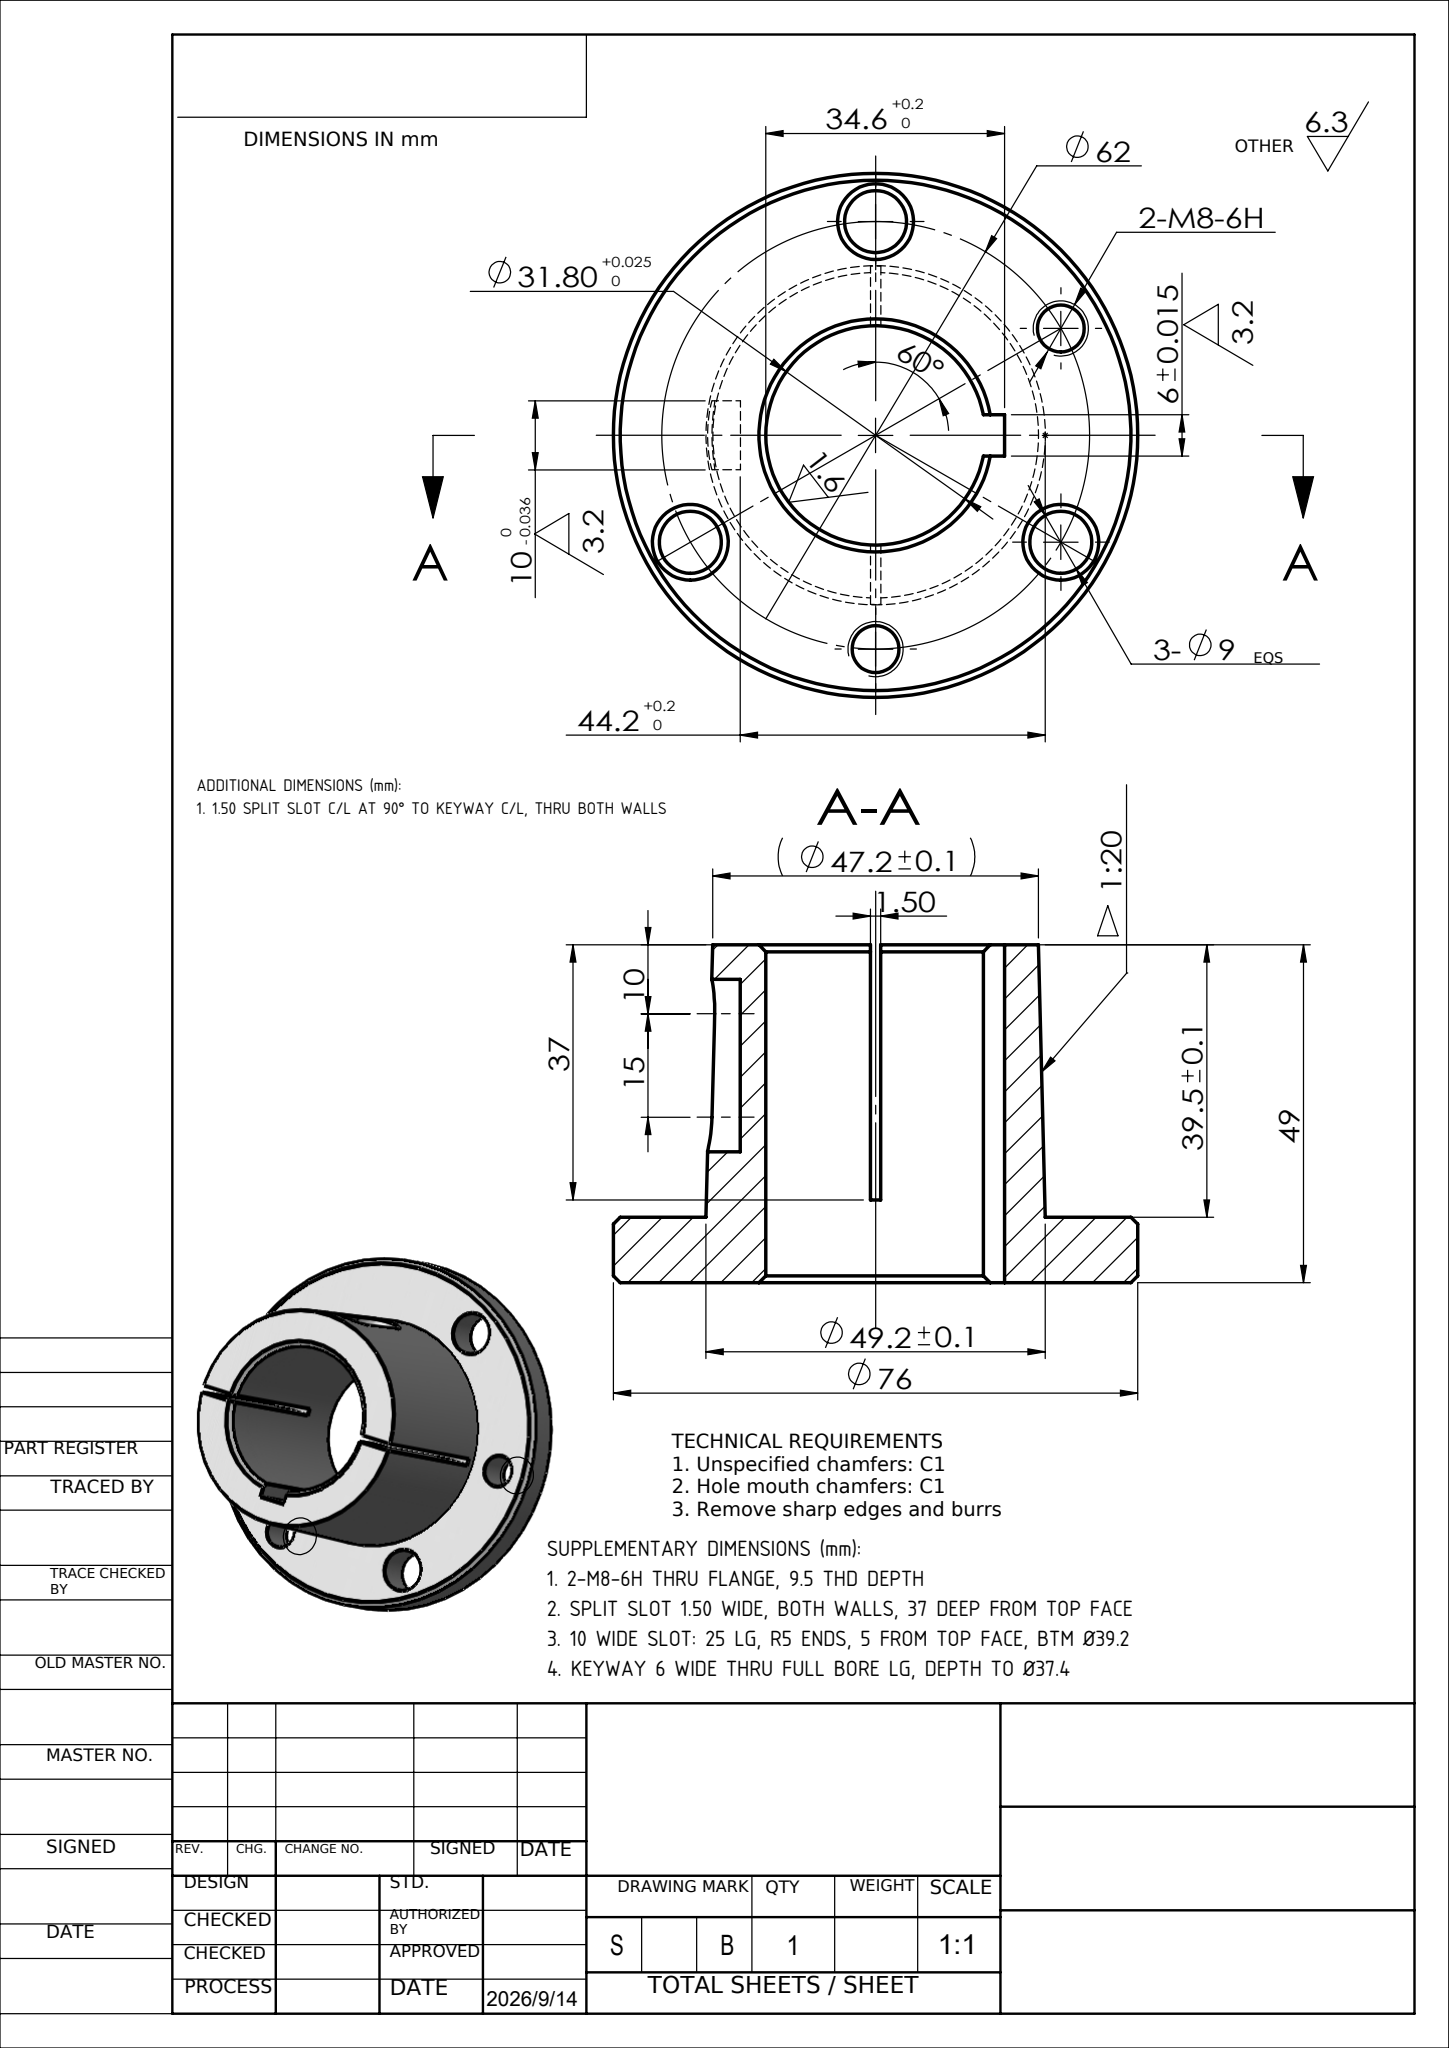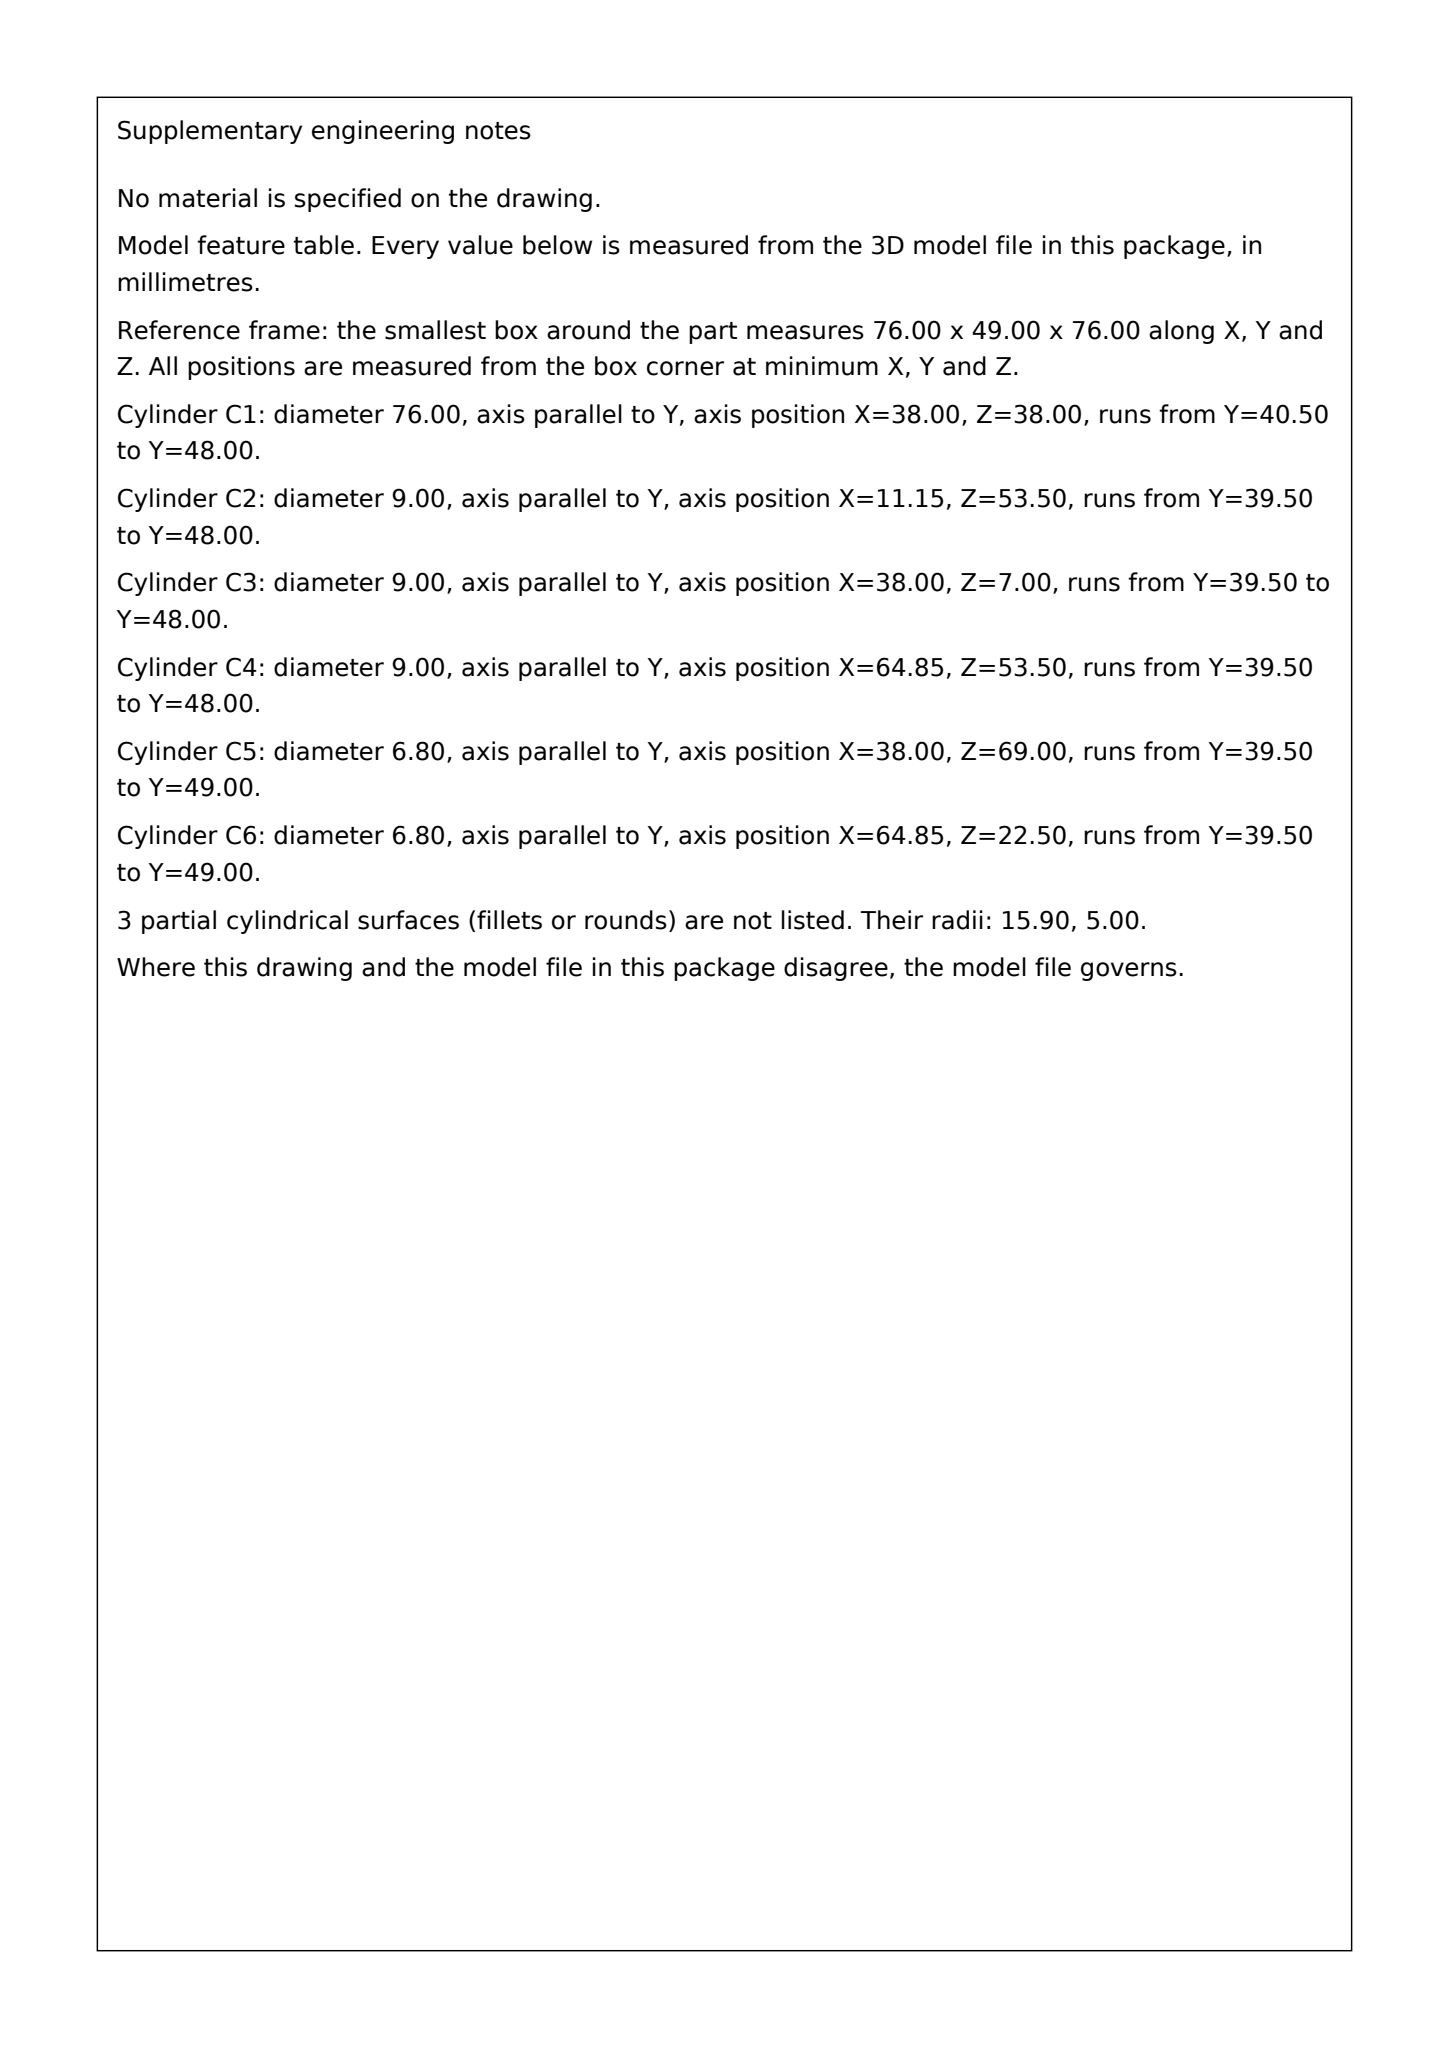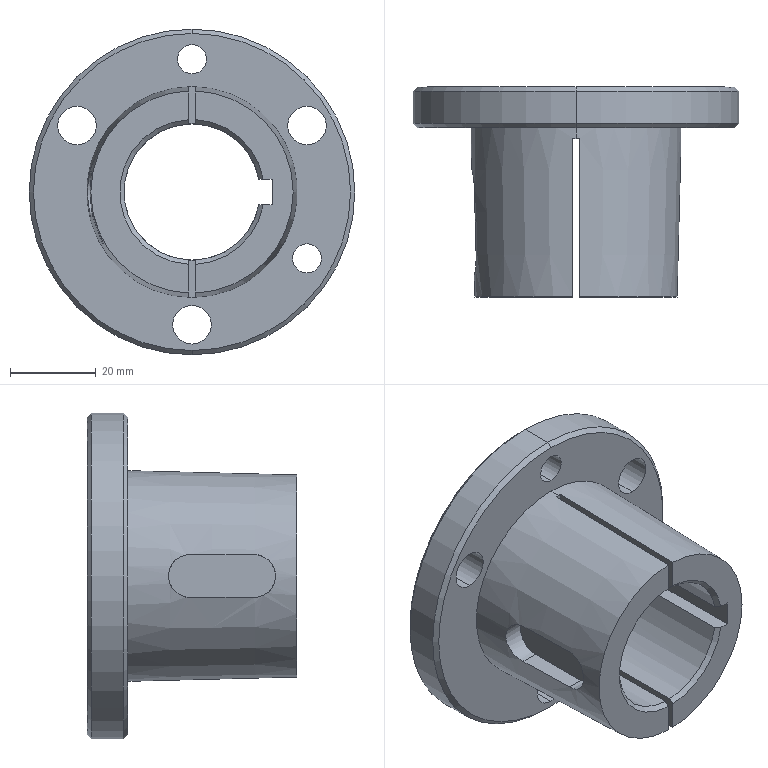Part | SolidWorks | mm | 1 solid | 51 faces | box 76 x 49 x 76 mm | volume 70647 mm3 | cone 18 | cylinder 17 | plane 16 | commonest cylinder face diameters 9 x6 6.8 x4 31.8 x3 76 x2 10 x2
build123d program:
from build123d import *

# Parameters (mm, degrees)
SKETCH2_W          = 13.691
SKETCH2_H          = 6
CUT_EXTRUDE1_DEPTH = 60
SKETCH3_W          = 1.5
SKETCH3_H          = 103.669
CUT_EXTRUDE2_DEPTH = 37
CHAMFER1_SIZE      = 1
SKETCH4_R          = 4.5
SKETCH4_R_2        = 1.75
CUT_EXTRUDE3_DEPTH = 24
M8_TAPPED_HOLE1_D  = 6.8
CHAMFER2_SIZE      = 1
CUT_EXTRUDE4_DEPTH = 5
CHAMFER3_SIZE      = 1


with BuildPart() as part:
    # Sketch1 → Revolve1 (revolve)
    with BuildSketch(Plane.XY, mode=Mode.PRIVATE) as revolve1_sk:
        Polygon((-15.9, 0), (-38, 0), (-38, -9.5), (-24.6, -9.5), (-23.6, -49), (-15.9, -49), align=None)
    revolve(revolve1_sk.sketch.rotate(Axis((0, 0, 0), (0, -1, 0)), 270), axis=Axis((0, 0, 0), (0, -1, 0)))

    # Sketch2 → Cut-Extrude1 (cut)
    with BuildSketch(Plane(origin=(0, 0, 0), x_dir=(1, 0, 0), z_dir=(0, 1, 0))):
        with Locations((11.854, 0)):
            Rectangle(SKETCH2_W, SKETCH2_H)
    extrude(amount=-CUT_EXTRUDE1_DEPTH, mode=Mode.SUBTRACT)

    # Sketch3 → Cut-Extrude2 (cut)
    with BuildSketch(Plane.XZ.offset(49)):
        with Locations((0, 5.408)):
            Rectangle(SKETCH3_W, SKETCH3_H)
    extrude(amount=-CUT_EXTRUDE2_DEPTH, mode=Mode.SUBTRACT)

    # Chamfer1
    chamfer1_edges = [part.edges().sort_by_distance(p)[0] for p in [
        (10.413, -49, -12.016),
        (-15.9, -49, 0),
        (10.413, -49, 12.016),
    ]]
    chamfer(chamfer1_edges, length=CHAMFER1_SIZE)

    # Sketch4 → Cut-Extrude3 (cut)
    with BuildSketch(Plane(origin=(0, 0, 0), x_dir=(1, 0, 0), z_dir=(0, 1, 0))):
        with Locations(Location((0, 31, 0), (0, 0, 270))):
            Circle(SKETCH4_R)
        with Locations(Location((26.847, -15.5, 0), (0, 0, 270))):
            Circle(SKETCH4_R)
        with Locations(Location((26.847, 15.5, 0), (0, 0, 270))):
            Circle(SKETCH4_R_2)
        with Locations(Location((0, -31, 0), (0, 0, 270))):
            Circle(SKETCH4_R_2)
        with Locations(Location((-26.847, -15.5, 0), (0, 0, 90))):
            Circle(SKETCH4_R)
    extrude(amount=-CUT_EXTRUDE3_DEPTH, mode=Mode.SUBTRACT)

    # M8 Tapped Hole1 (through all)
    with Locations(Plane(origin=(0, 0, 0), x_dir=(-1, 0, 0), z_dir=(0, 1, 0))):
        with Locations((0, 31), (-26.847, -15.5)):
            Hole(M8_TAPPED_HOLE1_D / 2)

    # Chamfer2
    chamfer2_edges = [part.edges().sort_by_distance(p)[0] for p in [
        (-15.9, 0, 0),
        (0, 0, -38),
        (0, -9.5, -38),
        (0, 0, -35.5),
        (26.847, 0, 11),
    ]]
    chamfer(chamfer2_edges, length=CHAMFER2_SIZE)

    # Sketch7 → Cut-Extrude4 (cut)
    with BuildSketch(Plane(origin=(-19.6, 0, 0), x_dir=(0, 0, -1), z_dir=(1, 0, 0))):
        with BuildLine():
            Line((5, -24), (5, -39))
            ThreePointArc((5, -39), (0, -44), (-5, -39))
            Line((-5, -39), (-5, -24))
            ThreePointArc((-5, -24), (0, -19), (5, -24))
        make_face()
    extrude(amount=-CUT_EXTRUDE4_DEPTH, mode=Mode.SUBTRACT)

    # Chamfer3
    chamfer3_edges = [part.edges().sort_by_distance(p)[0] for p in [
        (-26.847, 0, 20),
    ]]
    chamfer(chamfer3_edges, length=CHAMFER3_SIZE)


solid = part.part